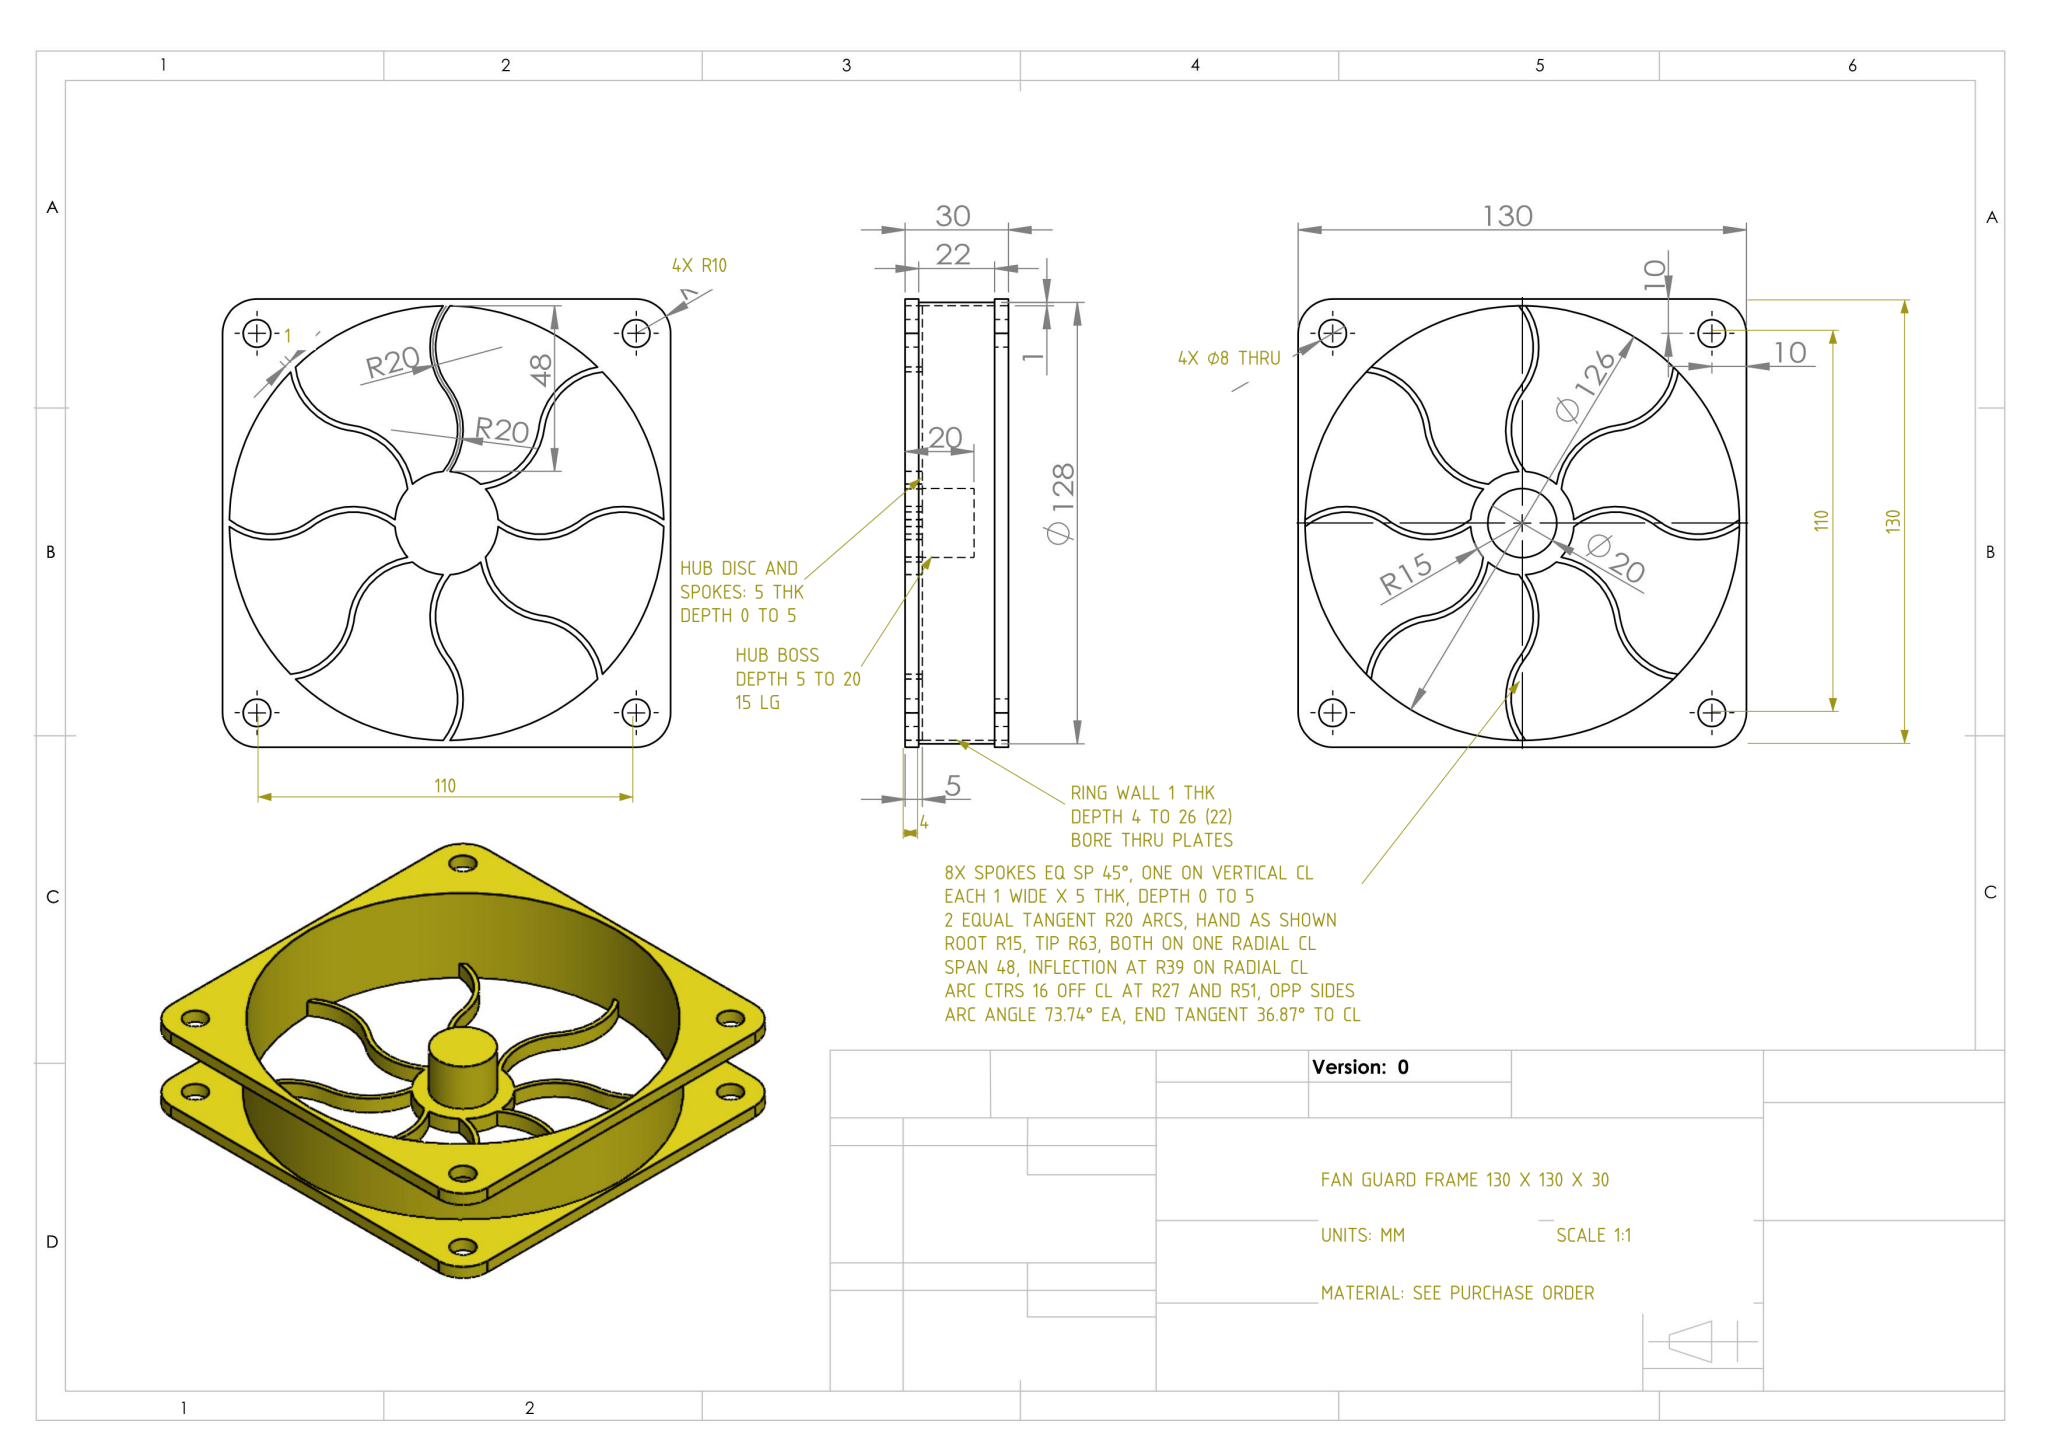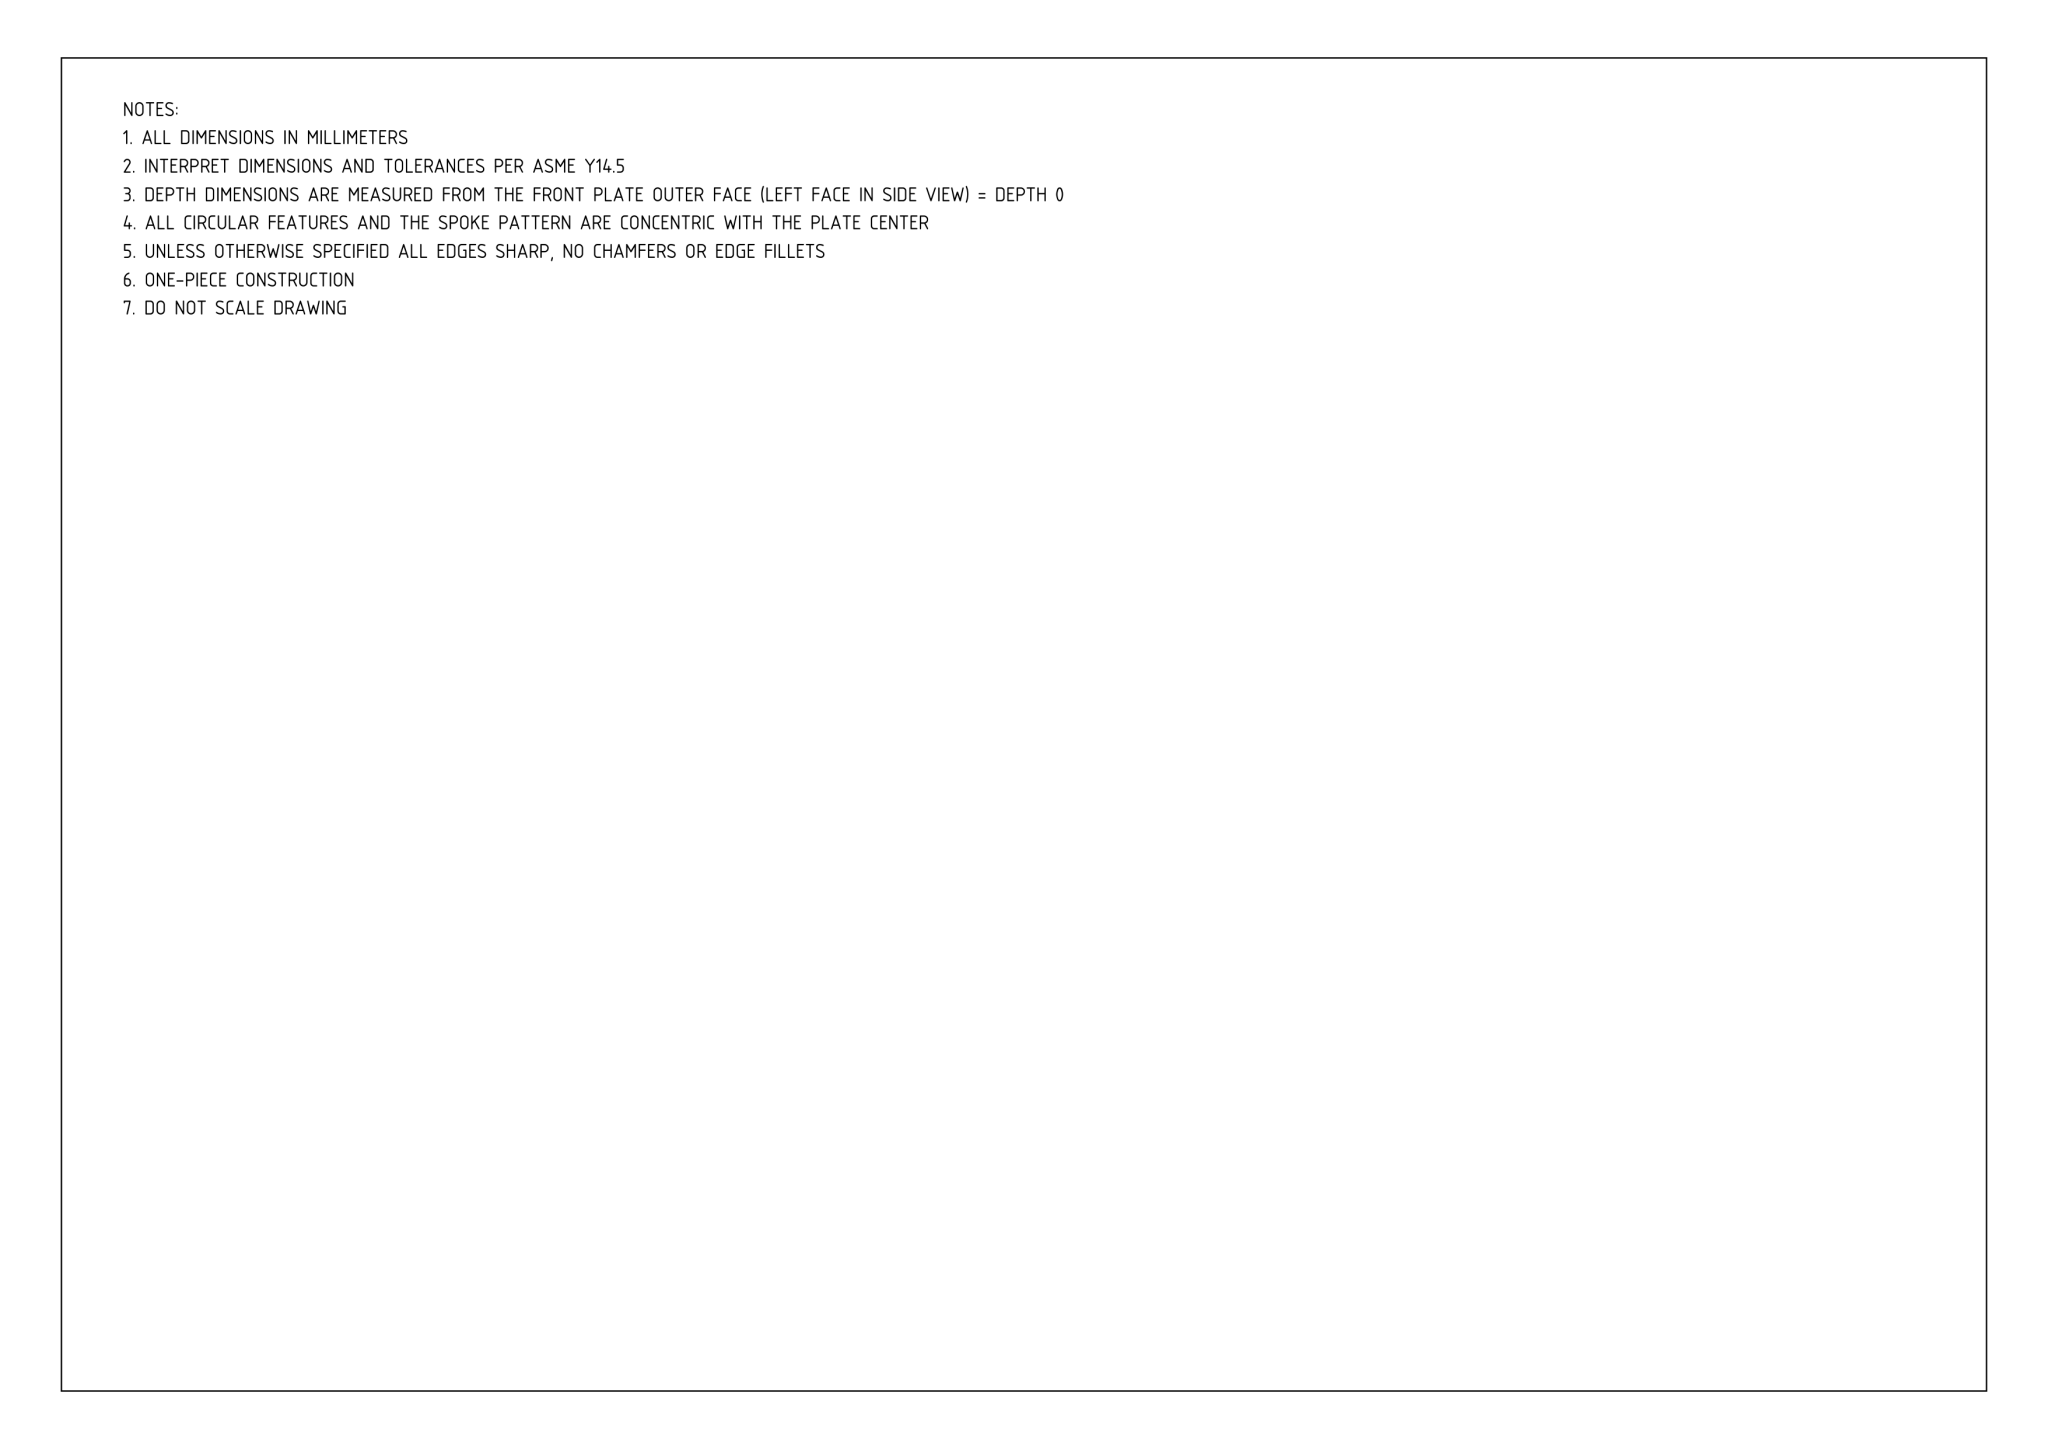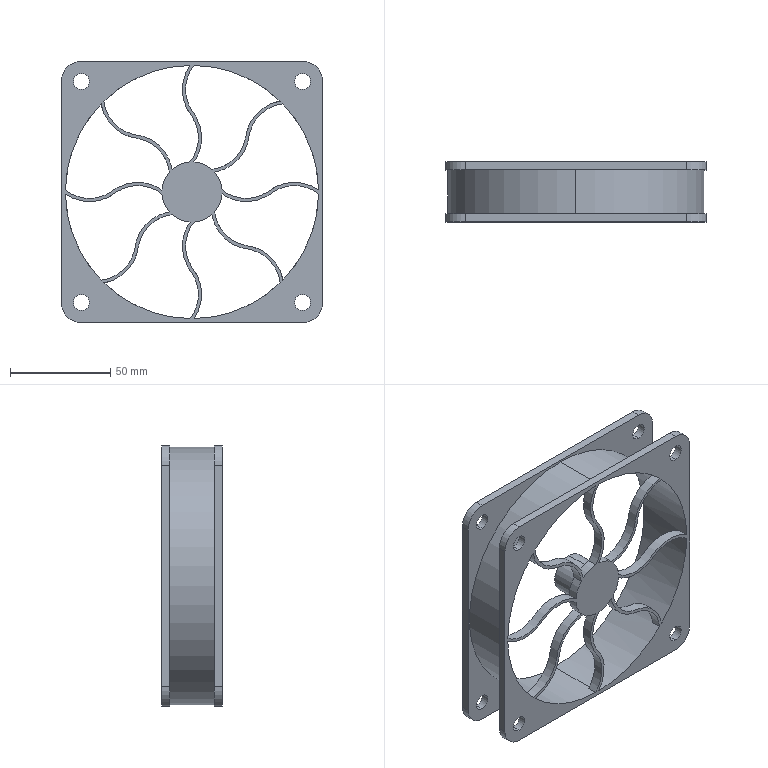Part | NX | mm | 1 solid | 68 faces | box 130 x 30 x 130 mm | volume 53497 mm3 | cylinder 38 | spline 16 | plane 14 | commonest cylinder face diameters 8 x16 20 x10 30 x8 128 x2 126 x2